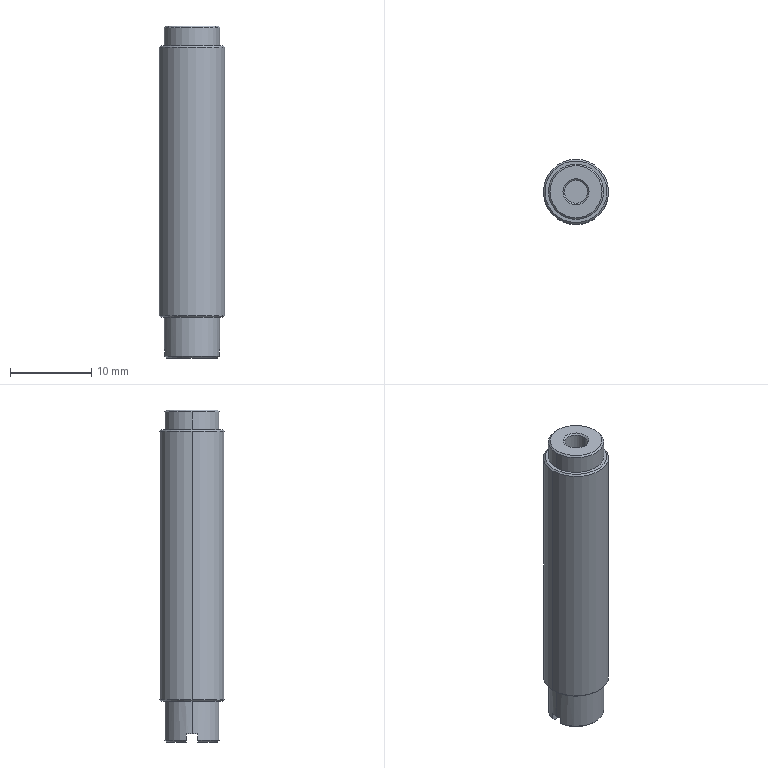Component | SolidWorks | F-YBXFJFA-RB0806-1_F-YBXFJFA-RB0806_Rb-Body-1 | 1 solid | 30 faces | box 8 x 8 x 40.8 mm | volume 1724 mm3 | cone 10 | cylinder 10 | plane 10 | commonest cylinder face diameters 6.8 x4 4.8 x2 2.8 x2 8 x2
build123d program:
from build123d import *

# Parameters (mm, degrees)
SKETCH1_R             = 4
BASE_EXTRUDE_DEPTH    = 20.4
SKETCH2_R             = 4
SKETCH2_R_2           = 3.4
FRONTNOTCH_DEPTH      = 2.4
REARNOTCH_START       = -5
SKETCH3_R             = 4
SKETCH3_R_2           = 3.4
REARNOTCH_DEPTH       = 5
SKETCH4_R             = 1.4
SHOCKHOLE_DEPTH       = 15
SKETCH5_R             = 2.4
STROKECHAMBER_DEPTH   = 10
CHAMFER1_SIZE         = 0.2
BLADENOTCH_DEPTH      = 22.17
BLADENOTCH_DEPTH_BACK = 22.17
SKETCH7_W             = 1
SKETCH7_H             = 1.4


with BuildPart() as part:
    # Sketch1 → Base-Extrude (new, symmetric)
    with BuildSketch(Plane.XY):
        Circle(SKETCH1_R)
    extrude(amount=BASE_EXTRUDE_DEPTH, both=True)

    # Sketch2 → FrontNotch (cut)
    with BuildSketch(Plane.XY.offset(20.4)):
        Circle(SKETCH2_R)
        Circle(SKETCH2_R_2, mode=Mode.SUBTRACT)
    extrude(amount=-FRONTNOTCH_DEPTH, mode=Mode.SUBTRACT)

    # Sketch3 → RearNotch (cut)
    with BuildSketch(Plane(origin=(0, 0, -20.4), x_dir=(-1, 0, 0), z_dir=(0, 0, -1)).offset(REARNOTCH_START)):
        with Locations(Location((0, 0, 0), (0, 0, 180))):
            Circle(SKETCH3_R)
        with Locations(Location((0, 0, 0), (0, 0, 180))):
            Circle(SKETCH3_R_2, mode=Mode.SUBTRACT)
    extrude(amount=REARNOTCH_DEPTH, mode=Mode.SUBTRACT)

    # Sketch4 → ShockHole (cut)
    with BuildSketch(Plane.XY.offset(20.4)):
        Circle(SKETCH4_R)
    extrude(amount=-SHOCKHOLE_DEPTH, mode=Mode.SUBTRACT)

    # Sketch5 → StrokeChamber (cut)
    with BuildSketch(Plane.XY.offset(5.4)):
        Circle(SKETCH5_R)
    extrude(amount=STROKECHAMBER_DEPTH, mode=Mode.SUBTRACT)

    # Chamfer1
    chamfer1_edges = [part.edges().sort_by_distance(p)[0] for p in [
        (-4, 0, -15.4),
        (-3.4, 0, -20.4),
        (-1.4, 0, 20.4),
        (-4, 0, 18),
        (-3.4, 0, 20.4),
    ]]
    chamfer(chamfer1_edges, length=CHAMFER1_SIZE)

    # Sketch7 → BladeNotch (cut, two sides: drawn at the far end of the back side and taken through both)
    with BuildSketch(Plane(origin=(0, 0, 0), x_dir=(0, 0, -1), z_dir=(1, 0, 0)).offset(-BLADENOTCH_DEPTH_BACK)):
        with Locations((19.9, 0)):
            Rectangle(SKETCH7_W, SKETCH7_H)
    extrude(amount=BLADENOTCH_DEPTH + BLADENOTCH_DEPTH_BACK, mode=Mode.SUBTRACT)


solid = part.part

# Placed as in the assembly
solid = solid.moved(Location((272.305, 309.175, 53.079), (0, 0, 0)))
STEP:
#1=CARTESIAN_POINT('',(10.571,12.172,1.483));
#2=VERTEX_POINT('',#1);
#3=CARTESIAN_POINT('',(10.87,12.172,1.483));
#4=VERTEX_POINT('',#3);
#5=CARTESIAN_POINT('',(10.721,12.172,1.483));
#6=DIRECTION('',(0.,0.,-1.));
#7=DIRECTION('',(1.,0.,0.));
#8=AXIS2_PLACEMENT_3D('',#5,#6,#7);
#9=CIRCLE('',#8,0.1496);
#10=EDGE_CURVE('',#2,#4,#9,.T.);
#11=ORIENTED_EDGE('',*,*,#10,.F.);
#12=CARTESIAN_POINT('',(10.563,12.172,1.491));
#13=VERTEX_POINT('',#12);
#14=CARTESIAN_POINT('',(10.571,12.172,1.483));
#15=DIRECTION('',(-0.7071,0.,0.7071));
#16=VECTOR('',#15,39.37);
#17=LINE('',#14,#16);
#18=EDGE_CURVE('',#2,#13,#17,.T.);
#19=ORIENTED_EDGE('',*,*,#18,.T.);
#20=CARTESIAN_POINT('',(10.878,12.172,1.491));
#21=VERTEX_POINT('',#20);
#22=CARTESIAN_POINT('',(10.721,12.172,1.491));
#23=DIRECTION('',(0.,0.,1.));
#24=DIRECTION('',(1.,0.,0.));
#25=AXIS2_PLACEMENT_3D('',#22,#23,#24);
#26=CIRCLE('',#25,0.1575);
#27=EDGE_CURVE('',#21,#13,#26,.T.);
#28=ORIENTED_EDGE('',*,*,#27,.F.);
#29=CARTESIAN_POINT('',(10.87,12.172,1.483));
#30=DIRECTION('',(0.7071,0.,0.7071));
#31=VECTOR('',#30,39.37);
#32=LINE('',#29,#31);
#33=EDGE_CURVE('',#4,#21,#32,.T.);
#34=ORIENTED_EDGE('',*,*,#33,.F.);
#35=EDGE_LOOP('',(#11,#19,#28,#34));
#36=FACE_OUTER_BOUND('',#35,.T.);
#37=CARTESIAN_POINT('',(10.721,12.172,1.483));
#38=DIRECTION('',(0.,0.,1.));
#39=DIRECTION('',(1.,0.,0.));
#40=AXIS2_PLACEMENT_3D('',#37,#38,#39);
#41=CONICAL_SURFACE('',#40,0.1496,0.7854);
#42=ADVANCED_FACE('',(#36),#41,.T.);
#43=CARTESIAN_POINT('',(10.87,12.172,2.798));
#44=VERTEX_POINT('',#43);
#45=CARTESIAN_POINT('',(10.571,12.172,2.798));
#46=VERTEX_POINT('',#45);
#47=CARTESIAN_POINT('',(10.721,12.172,2.798));
#48=DIRECTION('',(0.,0.,1.));
#49=DIRECTION('',(1.,0.,0.));
#50=AXIS2_PLACEMENT_3D('',#47,#48,#49);
#51=CIRCLE('',#50,0.1496);
#52=EDGE_CURVE('',#44,#46,#51,.T.);
#53=ORIENTED_EDGE('',*,*,#52,.F.);
#54=CARTESIAN_POINT('',(10.878,12.172,2.791));
#55=VERTEX_POINT('',#54);
#56=CARTESIAN_POINT('',(10.87,12.172,2.798));
#57=DIRECTION('',(0.7071,0.,-0.7071));
#58=VECTOR('',#57,39.37);
#59=LINE('',#56,#58);
#60=EDGE_CURVE('',#44,#55,#59,.T.);
#61=ORIENTED_EDGE('',*,*,#60,.T.);
#62=CARTESIAN_POINT('',(10.563,12.172,2.791));
#63=VERTEX_POINT('',#62);
#64=CARTESIAN_POINT('',(10.721,12.172,2.791));
#65=DIRECTION('',(0.,0.,-1.));
#66=DIRECTION('',(1.,0.,0.));
#67=AXIS2_PLACEMENT_3D('',#64,#65,#66);
#68=CIRCLE('',#67,0.1575);
#69=EDGE_CURVE('',#63,#55,#68,.T.);
#70=ORIENTED_EDGE('',*,*,#69,.F.);
#71=CARTESIAN_POINT('',(10.571,12.172,2.798));
#72=DIRECTION('',(-0.7071,0.,-0.7071));
#73=VECTOR('',#72,39.37);
#74=LINE('',#71,#73);
#75=EDGE_CURVE('',#46,#63,#74,.T.);
#76=ORIENTED_EDGE('',*,*,#75,.F.);
#77=EDGE_LOOP('',(#53,#61,#70,#76));
#78=FACE_OUTER_BOUND('',#77,.T.);
#79=CARTESIAN_POINT('',(10.721,12.172,2.798));
#80=DIRECTION('',(0.,0.,-1.));
#81=DIRECTION('',(-1.,0.,0.));
#82=AXIS2_PLACEMENT_3D('',#79,#80,#81);
#83=CONICAL_SURFACE('',#82,0.1496,0.7854);
#84=ADVANCED_FACE('',(#78),#83,.T.);
#85=CARTESIAN_POINT('',(10.847,12.172,2.893));
#86=VERTEX_POINT('',#85);
#87=CARTESIAN_POINT('',(10.595,12.172,2.893));
#88=VERTEX_POINT('',#87);
#89=CARTESIAN_POINT('',(10.721,12.172,2.893));
#90=DIRECTION('',(0.,0.,1.));
#91=DIRECTION('',(1.,0.,0.));
#92=AXIS2_PLACEMENT_3D('',#89,#90,#91);
#93=CIRCLE('',#92,0.126);
#94=EDGE_CURVE('',#86,#88,#93,.T.);
#95=ORIENTED_EDGE('',*,*,#94,.F.);
#96=CARTESIAN_POINT('',(10.855,12.172,2.885));
#97=VERTEX_POINT('',#96);
#98=CARTESIAN_POINT('',(10.847,12.172,2.893));
#99=DIRECTION('',(0.7071,0.,-0.7071));
#100=VECTOR('',#99,39.37);
#101=LINE('',#98,#100);
#102=EDGE_CURVE('',#86,#97,#101,.T.);
#103=ORIENTED_EDGE('',*,*,#102,.T.);
#104=CARTESIAN_POINT('',(10.587,12.172,2.885));
#105=VERTEX_POINT('',#104);
#106=CARTESIAN_POINT('',(10.721,12.172,2.885));
#107=DIRECTION('',(0.,0.,-1.));
#108=DIRECTION('',(1.,0.,0.));
#109=AXIS2_PLACEMENT_3D('',#106,#107,#108);
#110=CIRCLE('',#109,0.1339);
#111=EDGE_CURVE('',#105,#97,#110,.T.);
#112=ORIENTED_EDGE('',*,*,#111,.F.);
#113=CARTESIAN_POINT('',(10.595,12.172,2.893));
#114=DIRECTION('',(-0.7071,0.,-0.7071));
#115=VECTOR('',#114,39.37);
#116=LINE('',#113,#115);
#117=EDGE_CURVE('',#88,#105,#116,.T.);
#118=ORIENTED_EDGE('',*,*,#117,.F.);
#119=EDGE_LOOP('',(#95,#103,#112,#118));
#120=FACE_OUTER_BOUND('',#119,.T.);
#121=CARTESIAN_POINT('',(10.721,12.172,2.893));
#122=DIRECTION('',(0.,0.,-1.));
#123=DIRECTION('',(-1.,0.,0.));
#124=AXIS2_PLACEMENT_3D('',#121,#122,#123);
#125=CONICAL_SURFACE('',#124,0.126,0.7854);
#126=ADVANCED_FACE('',(#120),#125,.T.);
#127=CARTESIAN_POINT('',(10.666,12.172,2.885));
#128=VERTEX_POINT('',#127);
#129=CARTESIAN_POINT('',(10.776,12.172,2.885));
#130=VERTEX_POINT('',#129);
#131=CARTESIAN_POINT('',(10.721,12.172,2.885));
#132=DIRECTION('',(0.,0.,1.));
#133=DIRECTION('',(1.,0.,0.));
#134=AXIS2_PLACEMENT_3D('',#131,#132,#133);
#135=CIRCLE('',#134,0.05512);
#136=EDGE_CURVE('',#128,#130,#135,.T.);
#137=ORIENTED_EDGE('',*,*,#136,.F.);
#138=CARTESIAN_POINT('',(10.658,12.172,2.893));
#139=VERTEX_POINT('',#138);
#140=CARTESIAN_POINT('',(10.666,12.172,2.885));
#141=DIRECTION('',(-0.7071,0.,0.7071));
#142=VECTOR('',#141,39.37);
#143=LINE('',#140,#142);
#144=EDGE_CURVE('',#128,#139,#143,.T.);
#145=ORIENTED_EDGE('',*,*,#144,.T.);
#146=CARTESIAN_POINT('',(10.784,12.172,2.893));
#147=VERTEX_POINT('',#146);
#148=CARTESIAN_POINT('',(10.721,12.172,2.893));
#149=DIRECTION('',(0.,0.,-1.));
#150=DIRECTION('',(1.,0.,0.));
#151=AXIS2_PLACEMENT_3D('',#148,#149,#150);
#152=CIRCLE('',#151,0.06299);
#153=EDGE_CURVE('',#147,#139,#152,.T.);
#154=ORIENTED_EDGE('',*,*,#153,.F.);
#155=CARTESIAN_POINT('',(10.776,12.172,2.885));
#156=DIRECTION('',(0.7071,0.,0.7071));
#157=VECTOR('',#156,39.37);
#158=LINE('',#155,#157);
#159=EDGE_CURVE('',#130,#147,#158,.T.);
#160=ORIENTED_EDGE('',*,*,#159,.F.);
#161=EDGE_LOOP('',(#137,#145,#154,#160));
#162=FACE_OUTER_BOUND('',#161,.T.);
#163=CARTESIAN_POINT('',(10.721,12.172,2.885));
#164=DIRECTION('',(0.,0.,1.));
#165=DIRECTION('',(1.,0.,0.));
#166=AXIS2_PLACEMENT_3D('',#163,#164,#165);
#167=CONICAL_SURFACE('',#166,0.05512,0.7854);
#168=ADVANCED_FACE('',(#162),#167,.F.);
#169=CARTESIAN_POINT('',(10.626,12.172,2.696));
#170=VERTEX_POINT('',#169);
#171=CARTESIAN_POINT('',(10.815,12.172,2.696));
#172=VERTEX_POINT('',#171);
#173=CARTESIAN_POINT('',(10.721,12.172,2.696));
#174=DIRECTION('',(0.,0.,1.));
#175=DIRECTION('',(1.,0.,0.));
#176=AXIS2_PLACEMENT_3D('',#173,#174,#175);
#177=CIRCLE('',#176,0.09449);
#178=EDGE_CURVE('',#170,#172,#177,.T.);
#179=ORIENTED_EDGE('',*,*,#178,.T.);
#180=CARTESIAN_POINT('',(10.815,12.172,2.302));
#181=VERTEX_POINT('',#180);
#182=CARTESIAN_POINT('',(10.815,12.172,2.696));
#183=DIRECTION('',(0.,0.,-1.));
#184=VECTOR('',#183,39.37);
#185=LINE('',#182,#184);
#186=EDGE_CURVE('',#172,#181,#185,.T.);
#187=ORIENTED_EDGE('',*,*,#186,.T.);
#188=CARTESIAN_POINT('',(10.626,12.172,2.302));
#189=VERTEX_POINT('',#188);
#190=CARTESIAN_POINT('',(10.721,12.172,2.302));
#191=DIRECTION('',(0.,0.,1.));
#192=DIRECTION('',(1.,0.,0.));
#193=AXIS2_PLACEMENT_3D('',#190,#191,#192);
#194=CIRCLE('',#193,0.09449);
#195=EDGE_CURVE('',#189,#181,#194,.T.);
#196=ORIENTED_EDGE('',*,*,#195,.F.);
#197=CARTESIAN_POINT('',(10.626,12.172,2.696));
#198=DIRECTION('',(0.,0.,-1.));
#199=VECTOR('',#198,39.37);
#200=LINE('',#197,#199);
#201=EDGE_CURVE('',#170,#189,#200,.T.);
#202=ORIENTED_EDGE('',*,*,#201,.F.);
#203=EDGE_LOOP('',(#179,#187,#196,#202));
#204=FACE_OUTER_BOUND('',#203,.T.);
#205=CARTESIAN_POINT('',(10.721,12.172,2.696));
#206=DIRECTION('',(0.,0.,-1.));
#207=DIRECTION('',(-1.,0.,0.));
#208=AXIS2_PLACEMENT_3D('',#205,#206,#207);
#209=CYLINDRICAL_SURFACE('',#208,0.09449);
#210=ADVANCED_FACE('',(#204),#209,.F.);
#211=CARTESIAN_POINT('',(10.776,12.172,2.696));
#212=VERTEX_POINT('',#211);
#213=CARTESIAN_POINT('',(10.666,12.172,2.696));
#214=VERTEX_POINT('',#213);
#215=CARTESIAN_POINT('',(10.721,12.172,2.696));
#216=DIRECTION('',(0.,0.,-1.));
#217=DIRECTION('',(1.,0.,0.));
#218=AXIS2_PLACEMENT_3D('',#215,#216,#217);
#219=CIRCLE('',#218,0.05512);
#220=EDGE_CURVE('',#212,#214,#219,.T.);
#221=ORIENTED_EDGE('',*,*,#220,.T.);
#222=CARTESIAN_POINT('',(10.666,12.172,2.302));
#223=DIRECTION('',(0.,0.,1.));
#224=VECTOR('',#223,39.37);
#225=LINE('',#222,#224);
#226=EDGE_CURVE('',#214,#128,#225,.T.);
#227=ORIENTED_EDGE('',*,*,#226,.T.);
#228=ORIENTED_EDGE('',*,*,#136,.T.);
#229=CARTESIAN_POINT('',(10.776,12.172,2.302));
#230=DIRECTION('',(0.,0.,1.));
#231=VECTOR('',#230,39.37);
#232=LINE('',#229,#231);
#233=EDGE_CURVE('',#212,#130,#232,.T.);
#234=ORIENTED_EDGE('',*,*,#233,.F.);
#235=EDGE_LOOP('',(#221,#227,#228,#234));
#236=FACE_OUTER_BOUND('',#235,.T.);
#237=CARTESIAN_POINT('',(10.721,12.172,2.302));
#238=DIRECTION('',(0.,0.,1.));
#239=DIRECTION('',(1.,0.,0.));
#240=AXIS2_PLACEMENT_3D('',#237,#238,#239);
#241=CYLINDRICAL_SURFACE('',#240,0.05512);
#242=ADVANCED_FACE('',(#236),#241,.F.);
#243=CARTESIAN_POINT('',(10.587,12.172,1.483));
#244=VERTEX_POINT('',#243);
#245=CARTESIAN_POINT('',(10.855,12.172,1.483));
#246=VERTEX_POINT('',#245);
#247=CARTESIAN_POINT('',(10.721,12.172,1.483));
#248=DIRECTION('',(0.,0.,-1.));
#249=DIRECTION('',(1.,0.,0.));
#250=AXIS2_PLACEMENT_3D('',#247,#248,#249);
#251=CIRCLE('',#250,0.1339);
#252=EDGE_CURVE('',#244,#246,#251,.T.);
#253=ORIENTED_EDGE('',*,*,#252,.T.);
#254=CARTESIAN_POINT('',(10.855,12.172,1.326));
#255=VERTEX_POINT('',#254);
#256=CARTESIAN_POINT('',(10.855,12.172,3.244));
#257=DIRECTION('',(0.,0.,-1.));
#258=VECTOR('',#257,39.37);
#259=LINE('',#256,#258);
#260=EDGE_CURVE('',#246,#255,#259,.T.);
#261=ORIENTED_EDGE('',*,*,#260,.T.);
#262=CARTESIAN_POINT('',(10.852,12.2,1.326));
#263=VERTEX_POINT('',#262);
#264=CARTESIAN_POINT('',(10.721,12.172,1.326));
#265=DIRECTION('',(0.,0.,-1.));
#266=DIRECTION('',(1.,0.,0.));
#267=AXIS2_PLACEMENT_3D('',#264,#265,#266);
#268=CIRCLE('',#267,0.1339);
#269=EDGE_CURVE('',#263,#255,#268,.T.);
#270=ORIENTED_EDGE('',*,*,#269,.F.);
#271=CARTESIAN_POINT('',(10.852,12.2,1.294));
#272=VERTEX_POINT('',#271);
#273=CARTESIAN_POINT('',(10.852,12.2,3.244));
#274=DIRECTION('',(0.,0.,1.));
#275=VECTOR('',#274,39.37);
#276=LINE('',#273,#275);
#277=EDGE_CURVE('',#272,#263,#276,.T.);
#278=ORIENTED_EDGE('',*,*,#277,.F.);
#279=CARTESIAN_POINT('',(10.59,12.2,1.294));
#280=VERTEX_POINT('',#279);
#281=CARTESIAN_POINT('',(10.721,12.172,1.294));
#282=DIRECTION('',(0.,0.,1.));
#283=DIRECTION('',(1.,0.,0.));
#284=AXIS2_PLACEMENT_3D('',#281,#282,#283);
#285=CIRCLE('',#284,0.1339);
#286=EDGE_CURVE('',#272,#280,#285,.T.);
#287=ORIENTED_EDGE('',*,*,#286,.T.);
#288=CARTESIAN_POINT('',(10.59,12.2,1.326));
#289=VERTEX_POINT('',#288);
#290=CARTESIAN_POINT('',(10.59,12.2,3.244));
#291=DIRECTION('',(0.,0.,-1.));
#292=VECTOR('',#291,39.37);
#293=LINE('',#290,#292);
#294=EDGE_CURVE('',#289,#280,#293,.T.);
#295=ORIENTED_EDGE('',*,*,#294,.F.);
#296=CARTESIAN_POINT('',(10.587,12.172,1.326));
#297=VERTEX_POINT('',#296);
#298=CARTESIAN_POINT('',(10.721,12.172,1.326));
#299=DIRECTION('',(0.,0.,-1.));
#300=DIRECTION('',(1.,0.,0.));
#301=AXIS2_PLACEMENT_3D('',#298,#299,#300);
#302=CIRCLE('',#301,0.1339);
#303=EDGE_CURVE('',#297,#289,#302,.T.);
#304=ORIENTED_EDGE('',*,*,#303,.F.);
#305=CARTESIAN_POINT('',(10.587,12.172,3.244));
#306=DIRECTION('',(0.,0.,-1.));
#307=VECTOR('',#306,39.37);
#308=LINE('',#305,#307);
#309=EDGE_CURVE('',#244,#297,#308,.T.);
#310=ORIENTED_EDGE('',*,*,#309,.F.);
#311=EDGE_LOOP('',(#253,#261,#270,#278,#287,#295,#304,#310));
#312=FACE_OUTER_BOUND('',#311,.T.);
#313=CARTESIAN_POINT('',(10.721,12.172,3.244));
#314=DIRECTION('',(0.,0.,-1.));
#315=DIRECTION('',(-1.,0.,0.));
#316=AXIS2_PLACEMENT_3D('',#313,#314,#315);
#317=CYLINDRICAL_SURFACE('',#316,0.1339);
#318=ADVANCED_FACE('',(#312),#317,.T.);
#319=CARTESIAN_POINT('',(10.855,12.172,2.798));
#320=VERTEX_POINT('',#319);
#321=CARTESIAN_POINT('',(10.587,12.172,2.798));
#322=VERTEX_POINT('',#321);
#323=CARTESIAN_POINT('',(10.721,12.172,2.798));
#324=DIRECTION('',(0.,0.,1.));
#325=DIRECTION('',(1.,0.,0.));
#326=AXIS2_PLACEMENT_3D('',#323,#324,#325);
#327=CIRCLE('',#326,0.1339);
#328=EDGE_CURVE('',#320,#322,#327,.T.);
#329=ORIENTED_EDGE('',*,*,#328,.T.);
#330=CARTESIAN_POINT('',(10.587,12.172,2.798));
#331=DIRECTION('',(0.,0.,1.));
#332=VECTOR('',#331,39.37);
#333=LINE('',#330,#332);
#334=EDGE_CURVE('',#322,#105,#333,.T.);
#335=ORIENTED_EDGE('',*,*,#334,.T.);
#336=ORIENTED_EDGE('',*,*,#111,.T.);
#337=CARTESIAN_POINT('',(10.855,12.172,2.798));
#338=DIRECTION('',(0.,0.,1.));
#339=VECTOR('',#338,39.37);
#340=LINE('',#337,#339);
#341=EDGE_CURVE('',#320,#97,#340,.T.);
#342=ORIENTED_EDGE('',*,*,#341,.F.);
#343=EDGE_LOOP('',(#329,#335,#336,#342));
#344=FACE_OUTER_BOUND('',#343,.T.);
#345=CARTESIAN_POINT('',(10.721,12.172,2.798));
#346=DIRECTION('',(0.,0.,1.));
#347=DIRECTION('',(1.,0.,0.));
#348=AXIS2_PLACEMENT_3D('',#345,#346,#347);
#349=CYLINDRICAL_SURFACE('',#348,0.1339);
#350=ADVANCED_FACE('',(#344),#349,.T.);
#351=ORIENTED_EDGE('',*,*,#69,.T.);
#352=CARTESIAN_POINT('',(10.878,12.172,2.893));
#353=DIRECTION('',(0.,0.,-1.));
#354=VECTOR('',#353,39.37);
#355=LINE('',#352,#354);
#356=EDGE_CURVE('',#55,#21,#355,.T.);
#357=ORIENTED_EDGE('',*,*,#356,.T.);
#358=ORIENTED_EDGE('',*,*,#27,.T.);
#359=CARTESIAN_POINT('',(10.563,12.172,2.893));
#360=DIRECTION('',(0.,0.,-1.));
#361=VECTOR('',#360,39.37);
#362=LINE('',#359,#361);
#363=EDGE_CURVE('',#63,#13,#362,.T.);
#364=ORIENTED_EDGE('',*,*,#363,.F.);
#365=EDGE_LOOP('',(#351,#357,#358,#364));
#366=FACE_OUTER_BOUND('',#365,.T.);
#367=CARTESIAN_POINT('',(10.721,12.172,2.893));
#368=DIRECTION('',(0.,0.,-1.));
#369=DIRECTION('',(-1.,0.,0.));
#370=AXIS2_PLACEMENT_3D('',#367,#368,#369);
#371=CYLINDRICAL_SURFACE('',#370,0.1575);
#372=ADVANCED_FACE('',(#366),#371,.T.);
#373=CARTESIAN_POINT('',(10.844,12.145,1.287));
#374=VERTEX_POINT('',#373);
#375=CARTESIAN_POINT('',(10.598,12.145,1.287));
#376=VERTEX_POINT('',#375);
#377=CARTESIAN_POINT('',(10.721,12.172,1.287));
#378=DIRECTION('',(0.,0.,-1.));
#379=DIRECTION('',(1.,0.,0.));
#380=AXIS2_PLACEMENT_3D('',#377,#378,#379);
#381=CIRCLE('',#380,0.126);
#382=EDGE_CURVE('',#374,#376,#381,.T.);
#383=ORIENTED_EDGE('',*,*,#382,.T.);
#384=CARTESIAN_POINT('',(10.563,12.145,1.287));
#385=DIRECTION('',(1.,0.,0.));
#386=VECTOR('',#385,39.37);
#387=LINE('',#384,#386);
#388=EDGE_CURVE('',#376,#374,#387,.T.);
#389=ORIENTED_EDGE('',*,*,#388,.T.);
#390=EDGE_LOOP('',(#383,#389));
#391=FACE_OUTER_BOUND('',#390,.T.);
#392=CARTESIAN_POINT('',(10.721,12.172,1.287));
#393=DIRECTION('',(0.,0.,1.));
#394=DIRECTION('',(1.,0.,0.));
#395=AXIS2_PLACEMENT_3D('',#392,#393,#394);
#396=PLANE('',#395);
#397=ADVANCED_FACE('',(#391),#396,.F.);
#398=CARTESIAN_POINT('',(10.852,12.145,1.294));
#399=VERTEX_POINT('',#398);
#400=CARTESIAN_POINT('',(10.852,12.145,1.294));
#401=CARTESIAN_POINT('',(10.849,12.145,1.292));
#402=CARTESIAN_POINT('',(10.846,12.145,1.289));
#403=CARTESIAN_POINT('',(10.844,12.145,1.287));
#404=B_SPLINE_CURVE_WITH_KNOTS('',3,(#400,#401,#402,#403),.UNSPECIFIED.,.F.,.F.,(4,4),(0.005801,0.006087),.UNSPECIFIED.);
#405=EDGE_CURVE('',#399,#374,#404,.T.);
#406=ORIENTED_EDGE('',*,*,#405,.F.);
#407=CARTESIAN_POINT('',(10.59,12.145,1.294));
#408=VERTEX_POINT('',#407);
#409=CARTESIAN_POINT('',(10.721,12.172,1.294));
#410=DIRECTION('',(0.,0.,1.));
#411=DIRECTION('',(1.,0.,0.));
#412=AXIS2_PLACEMENT_3D('',#409,#410,#411);
#413=CIRCLE('',#412,0.1339);
#414=EDGE_CURVE('',#408,#399,#413,.T.);
#415=ORIENTED_EDGE('',*,*,#414,.F.);
#416=CARTESIAN_POINT('',(10.598,12.145,1.287));
#417=CARTESIAN_POINT('',(10.595,12.145,1.289));
#418=CARTESIAN_POINT('',(10.592,12.145,1.292));
#419=CARTESIAN_POINT('',(10.59,12.145,1.294));
#420=B_SPLINE_CURVE_WITH_KNOTS('',3,(#416,#417,#418,#419),.UNSPECIFIED.,.F.,.F.,(4,4),(0.01418,0.01446),.UNSPECIFIED.);
#421=EDGE_CURVE('',#376,#408,#420,.T.);
#422=ORIENTED_EDGE('',*,*,#421,.F.);
#423=ORIENTED_EDGE('',*,*,#382,.F.);
#424=EDGE_LOOP('',(#406,#415,#422,#423));
#425=FACE_OUTER_BOUND('',#424,.T.);
#426=CARTESIAN_POINT('',(10.721,12.172,1.287));
#427=DIRECTION('',(0.,0.,1.));
#428=DIRECTION('',(1.,0.,0.));
#429=AXIS2_PLACEMENT_3D('',#426,#427,#428);
#430=CONICAL_SURFACE('',#429,0.126,0.7854);
#431=ADVANCED_FACE('',(#425),#430,.T.);
#432=ORIENTED_EDGE('',*,*,#356,.F.);
#433=CARTESIAN_POINT('',(10.721,12.172,2.791));
#434=DIRECTION('',(0.,0.,-1.));
#435=DIRECTION('',(1.,0.,0.));
#436=AXIS2_PLACEMENT_3D('',#433,#434,#435);
#437=CIRCLE('',#436,0.1575);
#438=EDGE_CURVE('',#55,#63,#437,.T.);
#439=ORIENTED_EDGE('',*,*,#438,.T.);
#440=ORIENTED_EDGE('',*,*,#363,.T.);
#441=CARTESIAN_POINT('',(10.721,12.172,1.491));
#442=DIRECTION('',(0.,0.,1.));
#443=DIRECTION('',(1.,0.,0.));
#444=AXIS2_PLACEMENT_3D('',#441,#442,#443);
#445=CIRCLE('',#444,0.1575);
#446=EDGE_CURVE('',#13,#21,#445,.T.);
#447=ORIENTED_EDGE('',*,*,#446,.T.);
#448=EDGE_LOOP('',(#432,#439,#440,#447));
#449=FACE_OUTER_BOUND('',#448,.T.);
#450=CARTESIAN_POINT('',(10.721,12.172,2.893));
#451=DIRECTION('',(0.,0.,-1.));
#452=DIRECTION('',(-1.,0.,0.));
#453=AXIS2_PLACEMENT_3D('',#450,#451,#452);
#454=CYLINDRICAL_SURFACE('',#453,0.1575);
#455=ADVANCED_FACE('',(#449),#454,.T.);
#456=CARTESIAN_POINT('',(10.721,12.172,2.798));
#457=DIRECTION('',(0.,0.,1.));
#458=DIRECTION('',(1.,0.,0.));
#459=AXIS2_PLACEMENT_3D('',#456,#457,#458);
#460=CIRCLE('',#459,0.1496);
#461=EDGE_CURVE('',#46,#44,#460,.T.);
#462=ORIENTED_EDGE('',*,*,#461,.T.);
#463=ORIENTED_EDGE('',*,*,#52,.T.);
#464=EDGE_LOOP('',(#462,#463));
#465=FACE_OUTER_BOUND('',#464,.T.);
#466=ORIENTED_EDGE('',*,*,#328,.F.);
#467=CARTESIAN_POINT('',(10.721,12.172,2.798));
#468=DIRECTION('',(0.,0.,1.));
#469=DIRECTION('',(1.,0.,0.));
#470=AXIS2_PLACEMENT_3D('',#467,#468,#469);
#471=CIRCLE('',#470,0.1339);
#472=EDGE_CURVE('',#322,#320,#471,.T.);
#473=ORIENTED_EDGE('',*,*,#472,.F.);
#474=EDGE_LOOP('',(#466,#473));
#475=FACE_BOUND('',#474,.T.);
#476=CARTESIAN_POINT('',(10.721,12.172,2.798));
#477=DIRECTION('',(0.,0.,1.));
#478=DIRECTION('',(1.,0.,0.));
#479=AXIS2_PLACEMENT_3D('',#476,#477,#478);
#480=PLANE('',#479);
#481=ADVANCED_FACE('',(#465,#475),#480,.T.);
#482=ORIENTED_EDGE('',*,*,#334,.F.);
#483=ORIENTED_EDGE('',*,*,#472,.T.);
#484=ORIENTED_EDGE('',*,*,#341,.T.);
#485=CARTESIAN_POINT('',(10.721,12.172,2.885));
#486=DIRECTION('',(0.,0.,-1.));
#487=DIRECTION('',(1.,0.,0.));
#488=AXIS2_PLACEMENT_3D('',#485,#486,#487);
#489=CIRCLE('',#488,0.1339);
#490=EDGE_CURVE('',#97,#105,#489,.T.);
#491=ORIENTED_EDGE('',*,*,#490,.T.);
#492=EDGE_LOOP('',(#482,#483,#484,#491));
#493=FACE_OUTER_BOUND('',#492,.T.);
#494=CARTESIAN_POINT('',(10.721,12.172,2.798));
#495=DIRECTION('',(0.,0.,1.));
#496=DIRECTION('',(1.,0.,0.));
#497=AXIS2_PLACEMENT_3D('',#494,#495,#496);
#498=CYLINDRICAL_SURFACE('',#497,0.1339);
#499=ADVANCED_FACE('',(#493),#498,.T.);
#500=ORIENTED_EDGE('',*,*,#153,.T.);
#501=CARTESIAN_POINT('',(10.721,12.172,2.893));
#502=DIRECTION('',(0.,0.,-1.));
#503=DIRECTION('',(1.,0.,0.));
#504=AXIS2_PLACEMENT_3D('',#501,#502,#503);
#505=CIRCLE('',#504,0.06299);
#506=EDGE_CURVE('',#139,#147,#505,.T.);
#507=ORIENTED_EDGE('',*,*,#506,.T.);
#508=EDGE_LOOP('',(#500,#507));
#509=FACE_BOUND('',#508,.T.);
#510=CARTESIAN_POINT('',(10.721,12.172,2.893));
#511=DIRECTION('',(0.,0.,1.));
#512=DIRECTION('',(1.,0.,0.));
#513=AXIS2_PLACEMENT_3D('',#510,#511,#512);
#514=CIRCLE('',#513,0.126);
#515=EDGE_CURVE('',#88,#86,#514,.T.);
#516=ORIENTED_EDGE('',*,*,#515,.T.);
#517=ORIENTED_EDGE('',*,*,#94,.T.);
#518=EDGE_LOOP('',(#516,#517));
#519=FACE_OUTER_BOUND('',#518,.T.);
#520=CARTESIAN_POINT('',(10.721,12.172,2.893));
#521=DIRECTION('',(0.,0.,1.));
#522=DIRECTION('',(1.,0.,0.));
#523=AXIS2_PLACEMENT_3D('',#520,#521,#522);
#524=PLANE('',#523);
#525=ADVANCED_FACE('',(#509,#519),#524,.T.);
#526=ORIENTED_EDGE('',*,*,#260,.F.);
#527=CARTESIAN_POINT('',(10.721,12.172,1.483));
#528=DIRECTION('',(0.,0.,-1.));
#529=DIRECTION('',(1.,0.,0.));
#530=AXIS2_PLACEMENT_3D('',#527,#528,#529);
#531=CIRCLE('',#530,0.1339);
#532=EDGE_CURVE('',#246,#244,#531,.T.);
#533=ORIENTED_EDGE('',*,*,#532,.T.);
#534=ORIENTED_EDGE('',*,*,#309,.T.);
#535=CARTESIAN_POINT('',(10.59,12.145,1.326));
#536=VERTEX_POINT('',#535);
#537=CARTESIAN_POINT('',(10.721,12.172,1.326));
#538=DIRECTION('',(0.,0.,-1.));
#539=DIRECTION('',(1.,0.,0.));
#540=AXIS2_PLACEMENT_3D('',#537,#538,#539);
#541=CIRCLE('',#540,0.1339);
#542=EDGE_CURVE('',#536,#297,#541,.T.);
#543=ORIENTED_EDGE('',*,*,#542,.F.);
#544=CARTESIAN_POINT('',(10.59,12.145,3.244));
#545=DIRECTION('',(0.,0.,1.));
#546=VECTOR('',#545,39.37);
#547=LINE('',#544,#546);
#548=EDGE_CURVE('',#408,#536,#547,.T.);
#549=ORIENTED_EDGE('',*,*,#548,.F.);
#550=ORIENTED_EDGE('',*,*,#414,.T.);
#551=CARTESIAN_POINT('',(10.852,12.145,1.326));
#552=VERTEX_POINT('',#551);
#553=CARTESIAN_POINT('',(10.852,12.145,3.244));
#554=DIRECTION('',(0.,0.,-1.));
#555=VECTOR('',#554,39.37);
#556=LINE('',#553,#555);
#557=EDGE_CURVE('',#552,#399,#556,.T.);
#558=ORIENTED_EDGE('',*,*,#557,.F.);
#559=CARTESIAN_POINT('',(10.721,12.172,1.326));
#560=DIRECTION('',(0.,0.,-1.));
#561=DIRECTION('',(1.,0.,0.));
#562=AXIS2_PLACEMENT_3D('',#559,#560,#561);
#563=CIRCLE('',#562,0.1339);
#564=EDGE_CURVE('',#255,#552,#563,.T.);
#565=ORIENTED_EDGE('',*,*,#564,.F.);
#566=EDGE_LOOP('',(#526,#533,#534,#543,#549,#550,#558,#565));
#567=FACE_OUTER_BOUND('',#566,.T.);
#568=CARTESIAN_POINT('',(10.721,12.172,3.244));
#569=DIRECTION('',(0.,0.,-1.));
#570=DIRECTION('',(-1.,0.,0.));
#571=AXIS2_PLACEMENT_3D('',#568,#569,#570);
#572=CYLINDRICAL_SURFACE('',#571,0.1339);
#573=ADVANCED_FACE('',(#567),#572,.T.);
#574=CARTESIAN_POINT('',(10.721,12.172,1.483));
#575=DIRECTION('',(0.,0.,-1.));
#576=DIRECTION('',(1.,0.,0.));
#577=AXIS2_PLACEMENT_3D('',#574,#575,#576);
#578=CIRCLE('',#577,0.1496);
#579=EDGE_CURVE('',#4,#2,#578,.T.);
#580=ORIENTED_EDGE('',*,*,#579,.T.);
#581=ORIENTED_EDGE('',*,*,#10,.T.);
#582=EDGE_LOOP('',(#580,#581));
#583=FACE_OUTER_BOUND('',#582,.T.);
#584=ORIENTED_EDGE('',*,*,#252,.F.);
#585=ORIENTED_EDGE('',*,*,#532,.F.);
#586=EDGE_LOOP('',(#584,#585));
#587=FACE_BOUND('',#586,.T.);
#588=CARTESIAN_POINT('',(10.721,12.172,1.483));
#589=DIRECTION('',(0.,0.,1.));
#590=DIRECTION('',(1.,0.,0.));
#591=AXIS2_PLACEMENT_3D('',#588,#589,#590);
#592=PLANE('',#591);
#593=ADVANCED_FACE('',(#583,#587),#592,.F.);
#594=CARTESIAN_POINT('',(10.598,12.2,1.287));
#595=VERTEX_POINT('',#594);
#596=CARTESIAN_POINT('',(10.844,12.2,1.287));
#597=VERTEX_POINT('',#596);
#598=CARTESIAN_POINT('',(10.721,12.172,1.287));
#599=DIRECTION('',(0.,0.,-1.));
#600=DIRECTION('',(1.,0.,0.));
#601=AXIS2_PLACEMENT_3D('',#598,#599,#600);
#602=CIRCLE('',#601,0.126);
#603=EDGE_CURVE('',#595,#597,#602,.T.);
#604=ORIENTED_EDGE('',*,*,#603,.T.);
#605=CARTESIAN_POINT('',(10.563,12.2,1.287));
#606=DIRECTION('',(1.,0.,0.));
#607=VECTOR('',#606,39.37);
#608=LINE('',#605,#607);
#609=EDGE_CURVE('',#595,#597,#608,.T.);
#610=ORIENTED_EDGE('',*,*,#609,.F.);
#611=EDGE_LOOP('',(#604,#610));
#612=FACE_OUTER_BOUND('',#611,.T.);
#613=CARTESIAN_POINT('',(10.721,12.172,1.287));
#614=DIRECTION('',(0.,0.,1.));
#615=DIRECTION('',(1.,0.,0.));
#616=AXIS2_PLACEMENT_3D('',#613,#614,#615);
#617=PLANE('',#616);
#618=ADVANCED_FACE('',(#612),#617,.F.);
#619=ORIENTED_EDGE('',*,*,#226,.F.);
#620=CARTESIAN_POINT('',(10.721,12.172,2.696));
#621=DIRECTION('',(0.,0.,-1.));
#622=DIRECTION('',(1.,0.,0.));
#623=AXIS2_PLACEMENT_3D('',#620,#621,#622);
#624=CIRCLE('',#623,0.05512);
#625=EDGE_CURVE('',#214,#212,#624,.T.);
#626=ORIENTED_EDGE('',*,*,#625,.T.);
#627=ORIENTED_EDGE('',*,*,#233,.T.);
#628=CARTESIAN_POINT('',(10.721,12.172,2.885));
#629=DIRECTION('',(0.,0.,1.));
#630=DIRECTION('',(1.,0.,0.));
#631=AXIS2_PLACEMENT_3D('',#628,#629,#630);
#632=CIRCLE('',#631,0.05512);
#633=EDGE_CURVE('',#130,#128,#632,.T.);
#634=ORIENTED_EDGE('',*,*,#633,.T.);
#635=EDGE_LOOP('',(#619,#626,#627,#634));
#636=FACE_OUTER_BOUND('',#635,.T.);
#637=CARTESIAN_POINT('',(10.721,12.172,2.302));
#638=DIRECTION('',(0.,0.,1.));
#639=DIRECTION('',(1.,0.,0.));
#640=AXIS2_PLACEMENT_3D('',#637,#638,#639);
#641=CYLINDRICAL_SURFACE('',#640,0.05512);
#642=ADVANCED_FACE('',(#636),#641,.F.);
#643=ORIENTED_EDGE('',*,*,#178,.F.);
#644=CARTESIAN_POINT('',(10.721,12.172,2.696));
#645=DIRECTION('',(0.,0.,1.));
#646=DIRECTION('',(1.,0.,0.));
#647=AXIS2_PLACEMENT_3D('',#644,#645,#646);
#648=CIRCLE('',#647,0.09449);
#649=EDGE_CURVE('',#172,#170,#648,.T.);
#650=ORIENTED_EDGE('',*,*,#649,.F.);
#651=EDGE_LOOP('',(#643,#650));
#652=FACE_OUTER_BOUND('',#651,.T.);
#653=ORIENTED_EDGE('',*,*,#220,.F.);
#654=ORIENTED_EDGE('',*,*,#625,.F.);
#655=EDGE_LOOP('',(#653,#654));
#656=FACE_BOUND('',#655,.T.);
#657=CARTESIAN_POINT('',(10.721,12.172,2.696));
#658=DIRECTION('',(0.,0.,1.));
#659=DIRECTION('',(1.,0.,0.));
#660=AXIS2_PLACEMENT_3D('',#657,#658,#659);
#661=PLANE('',#660);
#662=ADVANCED_FACE('',(#652,#656),#661,.F.);
#663=ORIENTED_EDGE('',*,*,#186,.F.);
#664=ORIENTED_EDGE('',*,*,#649,.T.);
#665=ORIENTED_EDGE('',*,*,#201,.T.);
#666=CARTESIAN_POINT('',(10.721,12.172,2.302));
#667=DIRECTION('',(0.,0.,1.));
#668=DIRECTION('',(1.,0.,0.));
#669=AXIS2_PLACEMENT_3D('',#666,#667,#668);
#670=CIRCLE('',#669,0.09449);
#671=EDGE_CURVE('',#181,#189,#670,.T.);
#672=ORIENTED_EDGE('',*,*,#671,.F.);
#673=EDGE_LOOP('',(#663,#664,#665,#672));
#674=FACE_OUTER_BOUND('',#673,.T.);
#675=CARTESIAN_POINT('',(10.721,12.172,2.696));
#676=DIRECTION('',(0.,0.,-1.));
#677=DIRECTION('',(-1.,0.,0.));
#678=AXIS2_PLACEMENT_3D('',#675,#676,#677);
#679=CYLINDRICAL_SURFACE('',#678,0.09449);
#680=ADVANCED_FACE('',(#674),#679,.F.);
#681=ORIENTED_EDGE('',*,*,#195,.T.);
#682=ORIENTED_EDGE('',*,*,#671,.T.);
#683=EDGE_LOOP('',(#681,#682));
#684=FACE_OUTER_BOUND('',#683,.T.);
#685=CARTESIAN_POINT('',(10.721,12.172,2.302));
#686=DIRECTION('',(0.,0.,1.));
#687=DIRECTION('',(1.,0.,0.));
#688=AXIS2_PLACEMENT_3D('',#685,#686,#687);
#689=PLANE('',#688);
#690=ADVANCED_FACE('',(#684),#689,.T.);
#691=ORIENTED_EDGE('',*,*,#144,.F.);
#692=ORIENTED_EDGE('',*,*,#633,.F.);
#693=ORIENTED_EDGE('',*,*,#159,.T.);
#694=ORIENTED_EDGE('',*,*,#506,.F.);
#695=EDGE_LOOP('',(#691,#692,#693,#694));
#696=FACE_OUTER_BOUND('',#695,.T.);
#697=CARTESIAN_POINT('',(10.721,12.172,2.885));
#698=DIRECTION('',(0.,0.,1.));
#699=DIRECTION('',(1.,0.,0.));
#700=AXIS2_PLACEMENT_3D('',#697,#698,#699);
#701=CONICAL_SURFACE('',#700,0.05512,0.7854);
#702=ADVANCED_FACE('',(#696),#701,.F.);
#703=ORIENTED_EDGE('',*,*,#102,.F.);
#704=ORIENTED_EDGE('',*,*,#515,.F.);
#705=ORIENTED_EDGE('',*,*,#117,.T.);
#706=ORIENTED_EDGE('',*,*,#490,.F.);
#707=EDGE_LOOP('',(#703,#704,#705,#706));
#708=FACE_OUTER_BOUND('',#707,.T.);
#709=CARTESIAN_POINT('',(10.721,12.172,2.893));
#710=DIRECTION('',(0.,0.,-1.));
#711=DIRECTION('',(-1.,0.,0.));
#712=AXIS2_PLACEMENT_3D('',#709,#710,#711);
#713=CONICAL_SURFACE('',#712,0.126,0.7854);
#714=ADVANCED_FACE('',(#708),#713,.T.);
#715=ORIENTED_EDGE('',*,*,#60,.F.);
#716=ORIENTED_EDGE('',*,*,#461,.F.);
#717=ORIENTED_EDGE('',*,*,#75,.T.);
#718=ORIENTED_EDGE('',*,*,#438,.F.);
#719=EDGE_LOOP('',(#715,#716,#717,#718));
#720=FACE_OUTER_BOUND('',#719,.T.);
#721=CARTESIAN_POINT('',(10.721,12.172,2.798));
#722=DIRECTION('',(0.,0.,-1.));
#723=DIRECTION('',(-1.,0.,0.));
#724=AXIS2_PLACEMENT_3D('',#721,#722,#723);
#725=CONICAL_SURFACE('',#724,0.1496,0.7854);
#726=ADVANCED_FACE('',(#720),#725,.T.);
#727=CARTESIAN_POINT('',(10.59,12.2,1.294));
#728=CARTESIAN_POINT('',(10.592,12.2,1.292));
#729=CARTESIAN_POINT('',(10.595,12.2,1.289));
#730=CARTESIAN_POINT('',(10.598,12.2,1.287));
#731=B_SPLINE_CURVE_WITH_KNOTS('',3,(#727,#728,#729,#730),.UNSPECIFIED.,.F.,.F.,(4,4),(0.005801,0.006087),.UNSPECIFIED.);
#732=EDGE_CURVE('',#280,#595,#731,.T.);
#733=ORIENTED_EDGE('',*,*,#732,.F.);
#734=ORIENTED_EDGE('',*,*,#286,.F.);
#735=CARTESIAN_POINT('',(10.844,12.2,1.287));
#736=CARTESIAN_POINT('',(10.846,12.2,1.289));
#737=CARTESIAN_POINT('',(10.849,12.2,1.292));
#738=CARTESIAN_POINT('',(10.852,12.2,1.294));
#739=B_SPLINE_CURVE_WITH_KNOTS('',3,(#735,#736,#737,#738),.UNSPECIFIED.,.F.,.F.,(4,4),(0.01418,0.01446),.UNSPECIFIED.);
#740=EDGE_CURVE('',#597,#272,#739,.T.);
#741=ORIENTED_EDGE('',*,*,#740,.F.);
#742=ORIENTED_EDGE('',*,*,#603,.F.);
#743=EDGE_LOOP('',(#733,#734,#741,#742));
#744=FACE_OUTER_BOUND('',#743,.T.);
#745=CARTESIAN_POINT('',(10.721,12.172,1.287));
#746=DIRECTION('',(0.,0.,1.));
#747=DIRECTION('',(1.,0.,0.));
#748=AXIS2_PLACEMENT_3D('',#745,#746,#747);
#749=CONICAL_SURFACE('',#748,0.126,0.7854);
#750=ADVANCED_FACE('',(#744),#749,.T.);
#751=ORIENTED_EDGE('',*,*,#18,.F.);
#752=ORIENTED_EDGE('',*,*,#579,.F.);
#753=ORIENTED_EDGE('',*,*,#33,.T.);
#754=ORIENTED_EDGE('',*,*,#446,.F.);
#755=EDGE_LOOP('',(#751,#752,#753,#754));
#756=FACE_OUTER_BOUND('',#755,.T.);
#757=CARTESIAN_POINT('',(10.721,12.172,1.483));
#758=DIRECTION('',(0.,0.,1.));
#759=DIRECTION('',(1.,0.,0.));
#760=AXIS2_PLACEMENT_3D('',#757,#758,#759);
#761=CONICAL_SURFACE('',#760,0.1496,0.7854);
#762=ADVANCED_FACE('',(#756),#761,.T.);
#763=ORIENTED_EDGE('',*,*,#557,.T.);
#764=ORIENTED_EDGE('',*,*,#405,.T.);
#765=ORIENTED_EDGE('',*,*,#388,.F.);
#766=ORIENTED_EDGE('',*,*,#421,.T.);
#767=ORIENTED_EDGE('',*,*,#548,.T.);
#768=CARTESIAN_POINT('',(10.563,12.145,1.326));
#769=DIRECTION('',(1.,0.,0.));
#770=VECTOR('',#769,39.37);
#771=LINE('',#768,#770);
#772=EDGE_CURVE('',#536,#552,#771,.T.);
#773=ORIENTED_EDGE('',*,*,#772,.T.);
#774=EDGE_LOOP('',(#763,#764,#765,#766,#767,#773));
#775=FACE_OUTER_BOUND('',#774,.T.);
#776=CARTESIAN_POINT('',(10.563,12.145,1.287));
#777=DIRECTION('',(0.,-1.,-0.));
#778=DIRECTION('',(0.,0.,-1.));
#779=AXIS2_PLACEMENT_3D('',#776,#777,#778);
#780=PLANE('',#779);
#781=ADVANCED_FACE('',(#775),#780,.F.);
#782=ORIENTED_EDGE('',*,*,#542,.T.);
#783=ORIENTED_EDGE('',*,*,#303,.T.);
#784=CARTESIAN_POINT('',(10.563,12.2,1.326));
#785=DIRECTION('',(1.,0.,0.));
#786=VECTOR('',#785,39.37);
#787=LINE('',#784,#786);
#788=EDGE_CURVE('',#289,#263,#787,.T.);
#789=ORIENTED_EDGE('',*,*,#788,.T.);
#790=ORIENTED_EDGE('',*,*,#269,.T.);
#791=ORIENTED_EDGE('',*,*,#564,.T.);
#792=ORIENTED_EDGE('',*,*,#772,.F.);
#793=EDGE_LOOP('',(#782,#783,#789,#790,#791,#792));
#794=FACE_OUTER_BOUND('',#793,.T.);
#795=CARTESIAN_POINT('',(10.563,12.2,1.326));
#796=DIRECTION('',(0.,0.,1.));
#797=DIRECTION('',(1.,0.,0.));
#798=AXIS2_PLACEMENT_3D('',#795,#796,#797);
#799=PLANE('',#798);
#800=ADVANCED_FACE('',(#794),#799,.F.);
#801=ORIENTED_EDGE('',*,*,#294,.T.);
#802=ORIENTED_EDGE('',*,*,#732,.T.);
#803=ORIENTED_EDGE('',*,*,#609,.T.);
#804=ORIENTED_EDGE('',*,*,#740,.T.);
#805=ORIENTED_EDGE('',*,*,#277,.T.);
#806=ORIENTED_EDGE('',*,*,#788,.F.);
#807=EDGE_LOOP('',(#801,#802,#803,#804,#805,#806));
#808=FACE_OUTER_BOUND('',#807,.T.);
#809=CARTESIAN_POINT('',(10.563,12.2,1.287));
#810=DIRECTION('',(0.,1.,-0.));
#811=DIRECTION('',(0.,0.,1.));
#812=AXIS2_PLACEMENT_3D('',#809,#810,#811);
#813=PLANE('',#812);
#814=ADVANCED_FACE('',(#808),#813,.F.);
#815=CLOSED_SHELL('',(#42,#84,#126,#168,#210,#242,#318,#350,#372,#397,#431,#455,#481,#499,#525,#573,#593,#618,#642,#662,#680,#690,#702,#714,#726,#750,#762,#781,#800,#814));
#816=MANIFOLD_SOLID_BREP('',#815);
#817=CARTESIAN_POINT('',(0.,0.,0.));
#818=DIRECTION('',(0.,0.,1.));
#819=DIRECTION('',(1.,0.,0.));
#820=AXIS2_PLACEMENT_3D('',#817,#818,#819);
#821=(LENGTH_UNIT()NAMED_UNIT(*)SI_UNIT($,.METRE.));
#822=LENGTH_MEASURE_WITH_UNIT(LENGTH_MEASURE(0.0254),#821);
#823=DIMENSIONAL_EXPONENTS(1.,0.,0.,0.,0.,0.,0.);
#824=(CONVERSION_BASED_UNIT('',#822)LENGTH_UNIT()NAMED_UNIT(#823));
#825=UNCERTAINTY_MEASURE_WITH_UNIT(LENGTH_MEASURE(0.00001),#824,'','');
#826=(NAMED_UNIT(*)PLANE_ANGLE_UNIT()SI_UNIT($,.RADIAN.));
#827=(NAMED_UNIT(*)SI_UNIT($,.STERADIAN.)SOLID_ANGLE_UNIT());
#828=(GEOMETRIC_REPRESENTATION_CONTEXT(3)GLOBAL_UNCERTAINTY_ASSIGNED_CONTEXT((#825))GLOBAL_UNIT_ASSIGNED_CONTEXT((#824,#826,#827))REPRESENTATION_CONTEXT('',''));
#829=ADVANCED_BREP_SHAPE_REPRESENTATION('',(#816,#820),#828);
#830=COLOUR_RGB('',0.7922,0.8196,0.9333);
#831=FILL_AREA_STYLE_COLOUR('',#830);
#832=FILL_AREA_STYLE('',(#831));
#833=SURFACE_STYLE_FILL_AREA(#832);
#834=SURFACE_SIDE_STYLE('',(#833));
#835=SURFACE_STYLE_USAGE(.BOTH.,#834);
#836=PRESENTATION_STYLE_ASSIGNMENT((#835));
#837=STYLED_ITEM('',(#836),#816);
#838=PRESENTATION_LAYER_ASSIGNMENT('','',(#837));
#839=(LENGTH_UNIT()NAMED_UNIT(*)SI_UNIT($,.METRE.));
#840=LENGTH_MEASURE_WITH_UNIT(LENGTH_MEASURE(0.0254),#839);
#841=DIMENSIONAL_EXPONENTS(1.,0.,0.,0.,0.,0.,0.);
#842=(CONVERSION_BASED_UNIT('',#840)LENGTH_UNIT()NAMED_UNIT(#841));
#843=UNCERTAINTY_MEASURE_WITH_UNIT(LENGTH_MEASURE(0.00001),#842,'','');
#844=(NAMED_UNIT(*)PLANE_ANGLE_UNIT()SI_UNIT($,.RADIAN.));
#845=(NAMED_UNIT(*)SI_UNIT($,.STERADIAN.)SOLID_ANGLE_UNIT());
#846=(GEOMETRIC_REPRESENTATION_CONTEXT(3)GLOBAL_UNCERTAINTY_ASSIGNED_CONTEXT((#843))GLOBAL_UNIT_ASSIGNED_CONTEXT((#842,#844,#845))REPRESENTATION_CONTEXT('',''));
#847=MECHANICAL_DESIGN_GEOMETRIC_PRESENTATION_REPRESENTATION('',(#837),#846);